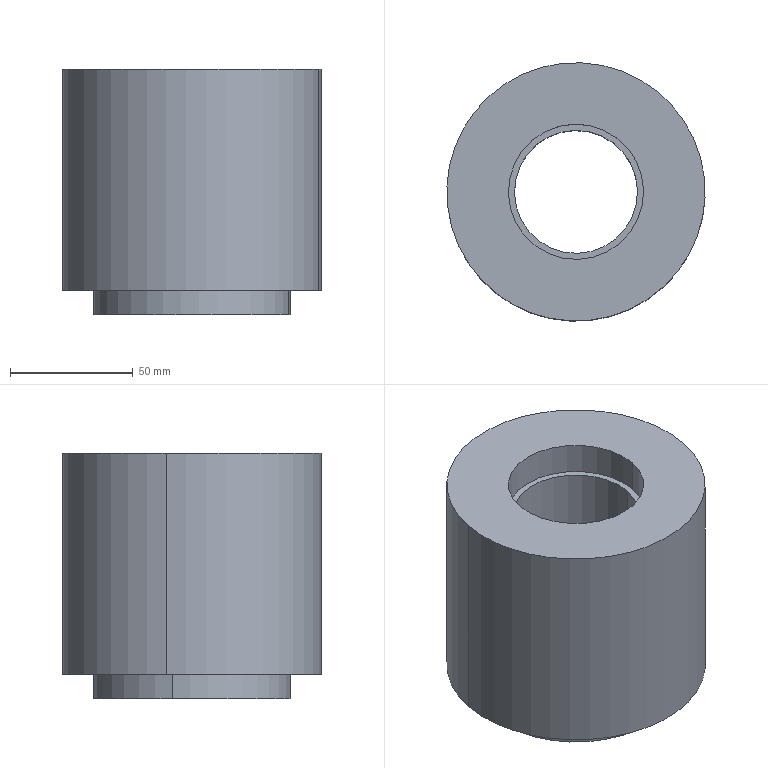Component | SolidWorks | -DrivenPulley-1 | 1 solid | 15 faces | box 105 x 105 x 100 mm | volume 622507 mm3 | cylinder 10 | plane 5 | commonest cylinder face diameters 55 x4 50 x2 80 x2 105 x2
build123d program:
from build123d import *


with BuildPart() as part:
    # Sketch1 → Revolve1 (revolve)
    with BuildSketch(Plane(origin=(0, 0, 0), x_dir=(1, 0, 0), z_dir=(0, 1, 0)), mode=Mode.PRIVATE) as revolve1_sk:
        Polygon((0, 52.5), (90, 52.5), (90, 40), (100, 40), (100, 27.5), (87, 27.5), (87, 25), (13, 25), (13, 27.5), (0, 27.5), align=None)
    revolve(revolve1_sk.sketch.rotate(Axis((-694.122, 0, 0), (1, 0, 0)), 180), axis=Axis((-694.122, 0, 0), (1, 0, 0)))


solid = part.part

# Placed as in the assembly
solid = solid.moved(Location((-130, 1094.5, 135), (0, 90, 0)))
STEP:
#1=COLOUR_RGB('',0.7922,0.8196,0.9333);
#2=FILL_AREA_STYLE_COLOUR('',#1);
#3=FILL_AREA_STYLE('',(#2));
#4=SURFACE_STYLE_FILL_AREA(#3);
#5=SURFACE_SIDE_STYLE('',(#4));
#6=SURFACE_STYLE_USAGE(.BOTH.,#5);
#7=PRESENTATION_STYLE_ASSIGNMENT((#6));
#8=CARTESIAN_POINT('',(-6.179,43.308,4.803));
#9=VERTEX_POINT('',#8);
#10=CARTESIAN_POINT('',(-4.057,42.873,4.803));
#11=VERTEX_POINT('',#10);
#12=CARTESIAN_POINT('',(-5.118,43.091,4.803));
#13=DIRECTION('',(0.,-0.,1.));
#14=DIRECTION('',(0.9797,-0.2007,-0.));
#15=AXIS2_PLACEMENT_3D('',#12,#13,#14);
#16=CIRCLE('',#15,1.083);
#17=EDGE_CURVE('',#9,#11,#16,.T.);
#18=ORIENTED_EDGE('',*,*,#17,.F.);
#19=CARTESIAN_POINT('',(-6.179,43.308,5.315));
#20=VERTEX_POINT('',#19);
#21=CARTESIAN_POINT('',(-6.179,43.308,32.643));
#22=DIRECTION('',(0.,-0.,1.));
#23=VECTOR('',#22,39.37);
#24=LINE('',#21,#23);
#25=EDGE_CURVE('',#9,#20,#24,.T.);
#26=ORIENTED_EDGE('',*,*,#25,.T.);
#27=CARTESIAN_POINT('',(-4.057,42.873,5.315));
#28=VERTEX_POINT('',#27);
#29=CARTESIAN_POINT('',(-5.118,43.091,5.315));
#30=DIRECTION('',(0.,-0.,1.));
#31=DIRECTION('',(0.9797,-0.2007,-0.));
#32=AXIS2_PLACEMENT_3D('',#29,#30,#31);
#33=CIRCLE('',#32,1.083);
#34=EDGE_CURVE('',#20,#28,#33,.T.);
#35=ORIENTED_EDGE('',*,*,#34,.T.);
#36=CARTESIAN_POINT('',(-4.057,42.873,32.643));
#37=DIRECTION('',(0.,-0.,1.));
#38=VECTOR('',#37,39.37);
#39=LINE('',#36,#38);
#40=EDGE_CURVE('',#11,#28,#39,.T.);
#41=ORIENTED_EDGE('',*,*,#40,.F.);
#42=EDGE_LOOP('',(#18,#26,#35,#41));
#43=FACE_OUTER_BOUND('',#42,.T.);
#44=CARTESIAN_POINT('',(-5.118,43.091,32.643));
#45=DIRECTION('',(0.,-0.,1.));
#46=DIRECTION('',(0.9797,-0.2007,0.));
#47=AXIS2_PLACEMENT_3D('',#44,#45,#46);
#48=CYLINDRICAL_SURFACE('',#47,1.083);
#49=ADVANCED_FACE('',(#43),#48,.F.);
#50=CARTESIAN_POINT('',(-6.082,43.288,1.89));
#51=VERTEX_POINT('',#50);
#52=CARTESIAN_POINT('',(-4.154,42.893,1.89));
#53=VERTEX_POINT('',#52);
#54=CARTESIAN_POINT('',(-5.118,43.091,1.89));
#55=DIRECTION('',(0.,-0.,1.));
#56=DIRECTION('',(0.9797,-0.2007,-0.));
#57=AXIS2_PLACEMENT_3D('',#54,#55,#56);
#58=CIRCLE('',#57,0.9843);
#59=EDGE_CURVE('',#51,#53,#58,.T.);
#60=ORIENTED_EDGE('',*,*,#59,.F.);
#61=CARTESIAN_POINT('',(-6.082,43.288,4.803));
#62=VERTEX_POINT('',#61);
#63=CARTESIAN_POINT('',(-6.082,43.288,32.643));
#64=DIRECTION('',(0.,-0.,1.));
#65=VECTOR('',#64,39.37);
#66=LINE('',#63,#65);
#67=EDGE_CURVE('',#51,#62,#66,.T.);
#68=ORIENTED_EDGE('',*,*,#67,.T.);
#69=CARTESIAN_POINT('',(-4.154,42.893,4.803));
#70=VERTEX_POINT('',#69);
#71=CARTESIAN_POINT('',(-5.118,43.091,4.803));
#72=DIRECTION('',(0.,-0.,1.));
#73=DIRECTION('',(0.9797,-0.2007,-0.));
#74=AXIS2_PLACEMENT_3D('',#71,#72,#73);
#75=CIRCLE('',#74,0.9843);
#76=EDGE_CURVE('',#62,#70,#75,.T.);
#77=ORIENTED_EDGE('',*,*,#76,.T.);
#78=CARTESIAN_POINT('',(-4.154,42.893,32.643));
#79=DIRECTION('',(0.,-0.,1.));
#80=VECTOR('',#79,39.37);
#81=LINE('',#78,#80);
#82=EDGE_CURVE('',#53,#70,#81,.T.);
#83=ORIENTED_EDGE('',*,*,#82,.F.);
#84=EDGE_LOOP('',(#60,#68,#77,#83));
#85=FACE_OUTER_BOUND('',#84,.T.);
#86=CARTESIAN_POINT('',(-5.118,43.091,32.643));
#87=DIRECTION('',(0.,-0.,1.));
#88=DIRECTION('',(0.9797,-0.2007,0.));
#89=AXIS2_PLACEMENT_3D('',#86,#87,#88);
#90=CYLINDRICAL_SURFACE('',#89,0.9843);
#91=ADVANCED_FACE('',(#85),#90,.F.);
#92=CARTESIAN_POINT('',(-6.179,43.308,1.378));
#93=VERTEX_POINT('',#92);
#94=CARTESIAN_POINT('',(-4.057,42.873,1.378));
#95=VERTEX_POINT('',#94);
#96=CARTESIAN_POINT('',(-5.118,43.091,1.378));
#97=DIRECTION('',(0.,-0.,1.));
#98=DIRECTION('',(0.9797,-0.2007,-0.));
#99=AXIS2_PLACEMENT_3D('',#96,#97,#98);
#100=CIRCLE('',#99,1.083);
#101=EDGE_CURVE('',#93,#95,#100,.T.);
#102=ORIENTED_EDGE('',*,*,#101,.F.);
#103=CARTESIAN_POINT('',(-6.179,43.308,1.89));
#104=VERTEX_POINT('',#103);
#105=CARTESIAN_POINT('',(-6.179,43.308,32.643));
#106=DIRECTION('',(0.,-0.,1.));
#107=VECTOR('',#106,39.37);
#108=LINE('',#105,#107);
#109=EDGE_CURVE('',#93,#104,#108,.T.);
#110=ORIENTED_EDGE('',*,*,#109,.T.);
#111=CARTESIAN_POINT('',(-4.057,42.873,1.89));
#112=VERTEX_POINT('',#111);
#113=CARTESIAN_POINT('',(-5.118,43.091,1.89));
#114=DIRECTION('',(0.,-0.,1.));
#115=DIRECTION('',(0.9797,-0.2007,-0.));
#116=AXIS2_PLACEMENT_3D('',#113,#114,#115);
#117=CIRCLE('',#116,1.083);
#118=EDGE_CURVE('',#104,#112,#117,.T.);
#119=ORIENTED_EDGE('',*,*,#118,.T.);
#120=CARTESIAN_POINT('',(-4.057,42.873,32.643));
#121=DIRECTION('',(0.,-0.,1.));
#122=VECTOR('',#121,39.37);
#123=LINE('',#120,#122);
#124=EDGE_CURVE('',#95,#112,#123,.T.);
#125=ORIENTED_EDGE('',*,*,#124,.F.);
#126=EDGE_LOOP('',(#102,#110,#119,#125));
#127=FACE_OUTER_BOUND('',#126,.T.);
#128=CARTESIAN_POINT('',(-5.118,43.091,32.643));
#129=DIRECTION('',(0.,-0.,1.));
#130=DIRECTION('',(0.9797,-0.2007,0.));
#131=AXIS2_PLACEMENT_3D('',#128,#129,#130);
#132=CYLINDRICAL_SURFACE('',#131,1.083);
#133=ADVANCED_FACE('',(#127),#132,.F.);
#134=CARTESIAN_POINT('',(-3.575,42.775,1.378));
#135=VERTEX_POINT('',#134);
#136=CARTESIAN_POINT('',(-6.661,43.407,1.378));
#137=VERTEX_POINT('',#136);
#138=CARTESIAN_POINT('',(-5.118,43.091,1.378));
#139=DIRECTION('',(0.,-0.,1.));
#140=DIRECTION('',(0.9797,-0.2007,-0.));
#141=AXIS2_PLACEMENT_3D('',#138,#139,#140);
#142=CIRCLE('',#141,1.575);
#143=EDGE_CURVE('',#135,#137,#142,.T.);
#144=ORIENTED_EDGE('',*,*,#143,.T.);
#145=CARTESIAN_POINT('',(-6.661,43.407,1.772));
#146=VERTEX_POINT('',#145);
#147=CARTESIAN_POINT('',(-6.661,43.407,32.643));
#148=DIRECTION('',(0.,-0.,1.));
#149=VECTOR('',#148,39.37);
#150=LINE('',#147,#149);
#151=EDGE_CURVE('',#137,#146,#150,.T.);
#152=ORIENTED_EDGE('',*,*,#151,.T.);
#153=CARTESIAN_POINT('',(-3.575,42.775,1.772));
#154=VERTEX_POINT('',#153);
#155=CARTESIAN_POINT('',(-5.118,43.091,1.772));
#156=DIRECTION('',(0.,-0.,1.));
#157=DIRECTION('',(0.9797,-0.2007,-0.));
#158=AXIS2_PLACEMENT_3D('',#155,#156,#157);
#159=CIRCLE('',#158,1.575);
#160=EDGE_CURVE('',#154,#146,#159,.T.);
#161=ORIENTED_EDGE('',*,*,#160,.F.);
#162=CARTESIAN_POINT('',(-3.575,42.775,32.643));
#163=DIRECTION('',(0.,-0.,1.));
#164=VECTOR('',#163,39.37);
#165=LINE('',#162,#164);
#166=EDGE_CURVE('',#135,#154,#165,.T.);
#167=ORIENTED_EDGE('',*,*,#166,.F.);
#168=EDGE_LOOP('',(#144,#152,#161,#167));
#169=FACE_OUTER_BOUND('',#168,.T.);
#170=CARTESIAN_POINT('',(-5.118,43.091,32.643));
#171=DIRECTION('',(0.,-0.,1.));
#172=DIRECTION('',(0.9797,-0.2007,0.));
#173=AXIS2_PLACEMENT_3D('',#170,#171,#172);
#174=CYLINDRICAL_SURFACE('',#173,1.575);
#175=ADVANCED_FACE('',(#169),#174,.T.);
#176=CARTESIAN_POINT('',(-3.093,42.676,1.772));
#177=VERTEX_POINT('',#176);
#178=CARTESIAN_POINT('',(-7.143,43.505,1.772));
#179=VERTEX_POINT('',#178);
#180=CARTESIAN_POINT('',(-5.118,43.091,1.772));
#181=DIRECTION('',(0.,-0.,1.));
#182=DIRECTION('',(0.9797,-0.2007,-0.));
#183=AXIS2_PLACEMENT_3D('',#180,#181,#182);
#184=CIRCLE('',#183,2.067);
#185=EDGE_CURVE('',#177,#179,#184,.T.);
#186=ORIENTED_EDGE('',*,*,#185,.T.);
#187=CARTESIAN_POINT('',(-7.143,43.505,5.315));
#188=VERTEX_POINT('',#187);
#189=CARTESIAN_POINT('',(-7.143,43.505,32.643));
#190=DIRECTION('',(0.,-0.,1.));
#191=VECTOR('',#190,39.37);
#192=LINE('',#189,#191);
#193=EDGE_CURVE('',#179,#188,#192,.T.);
#194=ORIENTED_EDGE('',*,*,#193,.T.);
#195=CARTESIAN_POINT('',(-3.093,42.676,5.315));
#196=VERTEX_POINT('',#195);
#197=CARTESIAN_POINT('',(-5.118,43.091,5.315));
#198=DIRECTION('',(0.,-0.,1.));
#199=DIRECTION('',(0.9797,-0.2007,-0.));
#200=AXIS2_PLACEMENT_3D('',#197,#198,#199);
#201=CIRCLE('',#200,2.067);
#202=EDGE_CURVE('',#196,#188,#201,.T.);
#203=ORIENTED_EDGE('',*,*,#202,.F.);
#204=CARTESIAN_POINT('',(-3.093,42.676,32.643));
#205=DIRECTION('',(0.,-0.,1.));
#206=VECTOR('',#205,39.37);
#207=LINE('',#204,#206);
#208=EDGE_CURVE('',#177,#196,#207,.T.);
#209=ORIENTED_EDGE('',*,*,#208,.F.);
#210=EDGE_LOOP('',(#186,#194,#203,#209));
#211=FACE_OUTER_BOUND('',#210,.T.);
#212=CARTESIAN_POINT('',(-5.118,43.091,32.643));
#213=DIRECTION('',(0.,-0.,1.));
#214=DIRECTION('',(0.9797,-0.2007,0.));
#215=AXIS2_PLACEMENT_3D('',#212,#213,#214);
#216=CYLINDRICAL_SURFACE('',#215,2.067);
#217=ADVANCED_FACE('',(#211),#216,.T.);
#218=CARTESIAN_POINT('',(-5.118,43.091,5.315));
#219=DIRECTION('',(0.,-0.,1.));
#220=DIRECTION('',(0.9797,-0.2007,-0.));
#221=AXIS2_PLACEMENT_3D('',#218,#219,#220);
#222=CIRCLE('',#221,1.083);
#223=EDGE_CURVE('',#28,#20,#222,.T.);
#224=ORIENTED_EDGE('',*,*,#223,.F.);
#225=ORIENTED_EDGE('',*,*,#34,.F.);
#226=EDGE_LOOP('',(#224,#225));
#227=FACE_BOUND('',#226,.T.);
#228=ORIENTED_EDGE('',*,*,#202,.T.);
#229=CARTESIAN_POINT('',(-5.118,43.091,5.315));
#230=DIRECTION('',(0.,-0.,1.));
#231=DIRECTION('',(0.9797,-0.2007,-0.));
#232=AXIS2_PLACEMENT_3D('',#229,#230,#231);
#233=CIRCLE('',#232,2.067);
#234=EDGE_CURVE('',#188,#196,#233,.T.);
#235=ORIENTED_EDGE('',*,*,#234,.T.);
#236=EDGE_LOOP('',(#228,#235));
#237=FACE_OUTER_BOUND('',#236,.T.);
#238=CARTESIAN_POINT('',(-6.179,43.308,5.315));
#239=DIRECTION('',(-0.,0.,-1.));
#240=DIRECTION('',(-0.9797,0.2007,0.));
#241=AXIS2_PLACEMENT_3D('',#238,#239,#240);
#242=PLANE('',#241);
#243=ADVANCED_FACE('',(#227,#237),#242,.F.);
#244=ORIENTED_EDGE('',*,*,#193,.F.);
#245=CARTESIAN_POINT('',(-5.118,43.091,1.772));
#246=DIRECTION('',(0.,-0.,1.));
#247=DIRECTION('',(0.9797,-0.2007,-0.));
#248=AXIS2_PLACEMENT_3D('',#245,#246,#247);
#249=CIRCLE('',#248,2.067);
#250=EDGE_CURVE('',#179,#177,#249,.T.);
#251=ORIENTED_EDGE('',*,*,#250,.T.);
#252=ORIENTED_EDGE('',*,*,#208,.T.);
#253=ORIENTED_EDGE('',*,*,#234,.F.);
#254=EDGE_LOOP('',(#244,#251,#252,#253));
#255=FACE_OUTER_BOUND('',#254,.T.);
#256=CARTESIAN_POINT('',(-5.118,43.091,32.643));
#257=DIRECTION('',(0.,-0.,1.));
#258=DIRECTION('',(0.9797,-0.2007,0.));
#259=AXIS2_PLACEMENT_3D('',#256,#257,#258);
#260=CYLINDRICAL_SURFACE('',#259,2.067);
#261=ADVANCED_FACE('',(#255),#260,.T.);
#262=ORIENTED_EDGE('',*,*,#185,.F.);
#263=ORIENTED_EDGE('',*,*,#250,.F.);
#264=EDGE_LOOP('',(#262,#263));
#265=FACE_OUTER_BOUND('',#264,.T.);
#266=ORIENTED_EDGE('',*,*,#160,.T.);
#267=CARTESIAN_POINT('',(-5.118,43.091,1.772));
#268=DIRECTION('',(0.,-0.,1.));
#269=DIRECTION('',(0.9797,-0.2007,-0.));
#270=AXIS2_PLACEMENT_3D('',#267,#268,#269);
#271=CIRCLE('',#270,1.575);
#272=EDGE_CURVE('',#146,#154,#271,.T.);
#273=ORIENTED_EDGE('',*,*,#272,.T.);
#274=EDGE_LOOP('',(#266,#273));
#275=FACE_BOUND('',#274,.T.);
#276=CARTESIAN_POINT('',(-7.143,43.505,1.772));
#277=DIRECTION('',(0.,-0.,1.));
#278=DIRECTION('',(0.9797,-0.2007,-0.));
#279=AXIS2_PLACEMENT_3D('',#276,#277,#278);
#280=PLANE('',#279);
#281=ADVANCED_FACE('',(#265,#275),#280,.F.);
#282=ORIENTED_EDGE('',*,*,#151,.F.);
#283=CARTESIAN_POINT('',(-5.118,43.091,1.378));
#284=DIRECTION('',(0.,-0.,1.));
#285=DIRECTION('',(0.9797,-0.2007,-0.));
#286=AXIS2_PLACEMENT_3D('',#283,#284,#285);
#287=CIRCLE('',#286,1.575);
#288=EDGE_CURVE('',#137,#135,#287,.T.);
#289=ORIENTED_EDGE('',*,*,#288,.T.);
#290=ORIENTED_EDGE('',*,*,#166,.T.);
#291=ORIENTED_EDGE('',*,*,#272,.F.);
#292=EDGE_LOOP('',(#282,#289,#290,#291));
#293=FACE_OUTER_BOUND('',#292,.T.);
#294=CARTESIAN_POINT('',(-5.118,43.091,32.643));
#295=DIRECTION('',(0.,-0.,1.));
#296=DIRECTION('',(0.9797,-0.2007,0.));
#297=AXIS2_PLACEMENT_3D('',#294,#295,#296);
#298=CYLINDRICAL_SURFACE('',#297,1.575);
#299=ADVANCED_FACE('',(#293),#298,.T.);
#300=ORIENTED_EDGE('',*,*,#143,.F.);
#301=ORIENTED_EDGE('',*,*,#288,.F.);
#302=EDGE_LOOP('',(#300,#301));
#303=FACE_OUTER_BOUND('',#302,.T.);
#304=CARTESIAN_POINT('',(-5.118,43.091,1.378));
#305=DIRECTION('',(0.,-0.,1.));
#306=DIRECTION('',(0.9797,-0.2007,-0.));
#307=AXIS2_PLACEMENT_3D('',#304,#305,#306);
#308=CIRCLE('',#307,1.083);
#309=EDGE_CURVE('',#95,#93,#308,.T.);
#310=ORIENTED_EDGE('',*,*,#309,.T.);
#311=ORIENTED_EDGE('',*,*,#101,.T.);
#312=EDGE_LOOP('',(#310,#311));
#313=FACE_BOUND('',#312,.T.);
#314=CARTESIAN_POINT('',(-6.661,43.407,1.378));
#315=DIRECTION('',(0.,-0.,1.));
#316=DIRECTION('',(0.9797,-0.2007,-0.));
#317=AXIS2_PLACEMENT_3D('',#314,#315,#316);
#318=PLANE('',#317);
#319=ADVANCED_FACE('',(#303,#313),#318,.F.);
#320=ORIENTED_EDGE('',*,*,#109,.F.);
#321=ORIENTED_EDGE('',*,*,#309,.F.);
#322=ORIENTED_EDGE('',*,*,#124,.T.);
#323=CARTESIAN_POINT('',(-5.118,43.091,1.89));
#324=DIRECTION('',(0.,-0.,1.));
#325=DIRECTION('',(0.9797,-0.2007,-0.));
#326=AXIS2_PLACEMENT_3D('',#323,#324,#325);
#327=CIRCLE('',#326,1.083);
#328=EDGE_CURVE('',#112,#104,#327,.T.);
#329=ORIENTED_EDGE('',*,*,#328,.T.);
#330=EDGE_LOOP('',(#320,#321,#322,#329));
#331=FACE_OUTER_BOUND('',#330,.T.);
#332=CARTESIAN_POINT('',(-5.118,43.091,32.643));
#333=DIRECTION('',(0.,-0.,1.));
#334=DIRECTION('',(0.9797,-0.2007,0.));
#335=AXIS2_PLACEMENT_3D('',#332,#333,#334);
#336=CYLINDRICAL_SURFACE('',#335,1.083);
#337=ADVANCED_FACE('',(#331),#336,.F.);
#338=ORIENTED_EDGE('',*,*,#328,.F.);
#339=ORIENTED_EDGE('',*,*,#118,.F.);
#340=EDGE_LOOP('',(#338,#339));
#341=FACE_OUTER_BOUND('',#340,.T.);
#342=CARTESIAN_POINT('',(-5.118,43.091,1.89));
#343=DIRECTION('',(0.,-0.,1.));
#344=DIRECTION('',(0.9797,-0.2007,-0.));
#345=AXIS2_PLACEMENT_3D('',#342,#343,#344);
#346=CIRCLE('',#345,0.9843);
#347=EDGE_CURVE('',#53,#51,#346,.T.);
#348=ORIENTED_EDGE('',*,*,#347,.T.);
#349=ORIENTED_EDGE('',*,*,#59,.T.);
#350=EDGE_LOOP('',(#348,#349));
#351=FACE_BOUND('',#350,.T.);
#352=CARTESIAN_POINT('',(-6.082,43.288,1.89));
#353=DIRECTION('',(0.,-0.,1.));
#354=DIRECTION('',(0.9797,-0.2007,-0.));
#355=AXIS2_PLACEMENT_3D('',#352,#353,#354);
#356=PLANE('',#355);
#357=ADVANCED_FACE('',(#341,#351),#356,.F.);
#358=ORIENTED_EDGE('',*,*,#67,.F.);
#359=ORIENTED_EDGE('',*,*,#347,.F.);
#360=ORIENTED_EDGE('',*,*,#82,.T.);
#361=CARTESIAN_POINT('',(-5.118,43.091,4.803));
#362=DIRECTION('',(0.,-0.,1.));
#363=DIRECTION('',(0.9797,-0.2007,-0.));
#364=AXIS2_PLACEMENT_3D('',#361,#362,#363);
#365=CIRCLE('',#364,0.9843);
#366=EDGE_CURVE('',#70,#62,#365,.T.);
#367=ORIENTED_EDGE('',*,*,#366,.T.);
#368=EDGE_LOOP('',(#358,#359,#360,#367));
#369=FACE_OUTER_BOUND('',#368,.T.);
#370=CARTESIAN_POINT('',(-5.118,43.091,32.643));
#371=DIRECTION('',(0.,-0.,1.));
#372=DIRECTION('',(0.9797,-0.2007,0.));
#373=AXIS2_PLACEMENT_3D('',#370,#371,#372);
#374=CYLINDRICAL_SURFACE('',#373,0.9843);
#375=ADVANCED_FACE('',(#369),#374,.F.);
#376=ORIENTED_EDGE('',*,*,#366,.F.);
#377=ORIENTED_EDGE('',*,*,#76,.F.);
#378=EDGE_LOOP('',(#376,#377));
#379=FACE_BOUND('',#378,.T.);
#380=CARTESIAN_POINT('',(-5.118,43.091,4.803));
#381=DIRECTION('',(0.,-0.,1.));
#382=DIRECTION('',(0.9797,-0.2007,-0.));
#383=AXIS2_PLACEMENT_3D('',#380,#381,#382);
#384=CIRCLE('',#383,1.083);
#385=EDGE_CURVE('',#11,#9,#384,.T.);
#386=ORIENTED_EDGE('',*,*,#385,.T.);
#387=ORIENTED_EDGE('',*,*,#17,.T.);
#388=EDGE_LOOP('',(#386,#387));
#389=FACE_OUTER_BOUND('',#388,.T.);
#390=CARTESIAN_POINT('',(-6.082,43.288,4.803));
#391=DIRECTION('',(-0.,0.,-1.));
#392=DIRECTION('',(-0.9797,0.2007,0.));
#393=AXIS2_PLACEMENT_3D('',#390,#391,#392);
#394=PLANE('',#393);
#395=ADVANCED_FACE('',(#379,#389),#394,.F.);
#396=ORIENTED_EDGE('',*,*,#25,.F.);
#397=ORIENTED_EDGE('',*,*,#385,.F.);
#398=ORIENTED_EDGE('',*,*,#40,.T.);
#399=ORIENTED_EDGE('',*,*,#223,.T.);
#400=EDGE_LOOP('',(#396,#397,#398,#399));
#401=FACE_OUTER_BOUND('',#400,.T.);
#402=CARTESIAN_POINT('',(-5.118,43.091,32.643));
#403=DIRECTION('',(0.,-0.,1.));
#404=DIRECTION('',(0.9797,-0.2007,0.));
#405=AXIS2_PLACEMENT_3D('',#402,#403,#404);
#406=CYLINDRICAL_SURFACE('',#405,1.083);
#407=ADVANCED_FACE('',(#401),#406,.F.);
#408=CLOSED_SHELL('',(#49,#91,#133,#175,#217,#243,#261,#281,#299,#319,#337,#357,#375,#395,#407));
#409=MANIFOLD_SOLID_BREP('',#408);
#410=STYLED_ITEM('',(#7),#409);
#411=(LENGTH_UNIT()NAMED_UNIT(*)SI_UNIT($,.METRE.));
#412=LENGTH_MEASURE_WITH_UNIT(LENGTH_MEASURE(0.0254),#411);
#413=DIMENSIONAL_EXPONENTS(1.,0.,0.,0.,0.,0.,0.);
#414=(CONVERSION_BASED_UNIT('',#412)LENGTH_UNIT()NAMED_UNIT(#413));
#415=UNCERTAINTY_MEASURE_WITH_UNIT(LENGTH_MEASURE(0.00001),#414,'','');
#416=(NAMED_UNIT(*)PLANE_ANGLE_UNIT()SI_UNIT($,.RADIAN.));
#417=(NAMED_UNIT(*)SI_UNIT($,.STERADIAN.)SOLID_ANGLE_UNIT());
#418=(GEOMETRIC_REPRESENTATION_CONTEXT(3)GLOBAL_UNCERTAINTY_ASSIGNED_CONTEXT((#415))GLOBAL_UNIT_ASSIGNED_CONTEXT((#414,#416,#417))REPRESENTATION_CONTEXT('',''));
#419=MECHANICAL_DESIGN_GEOMETRIC_PRESENTATION_REPRESENTATION('',(#410),#418);
#420=PRESENTATION_LAYER_ASSIGNMENT('','',(#410));
#421=CARTESIAN_POINT('',(0.,0.,0.));
#422=DIRECTION('',(0.,0.,1.));
#423=DIRECTION('',(1.,0.,0.));
#424=AXIS2_PLACEMENT_3D('',#421,#422,#423);
#425=(LENGTH_UNIT()NAMED_UNIT(*)SI_UNIT($,.METRE.));
#426=LENGTH_MEASURE_WITH_UNIT(LENGTH_MEASURE(0.0254),#425);
#427=DIMENSIONAL_EXPONENTS(1.,0.,0.,0.,0.,0.,0.);
#428=(CONVERSION_BASED_UNIT('',#426)LENGTH_UNIT()NAMED_UNIT(#427));
#429=UNCERTAINTY_MEASURE_WITH_UNIT(LENGTH_MEASURE(0.00001),#428,'','');
#430=(NAMED_UNIT(*)PLANE_ANGLE_UNIT()SI_UNIT($,.RADIAN.));
#431=(NAMED_UNIT(*)SI_UNIT($,.STERADIAN.)SOLID_ANGLE_UNIT());
#432=(GEOMETRIC_REPRESENTATION_CONTEXT(3)GLOBAL_UNCERTAINTY_ASSIGNED_CONTEXT((#429))GLOBAL_UNIT_ASSIGNED_CONTEXT((#428,#430,#431))REPRESENTATION_CONTEXT('',''));
#433=ADVANCED_BREP_SHAPE_REPRESENTATION('',(#409,#424),#432);